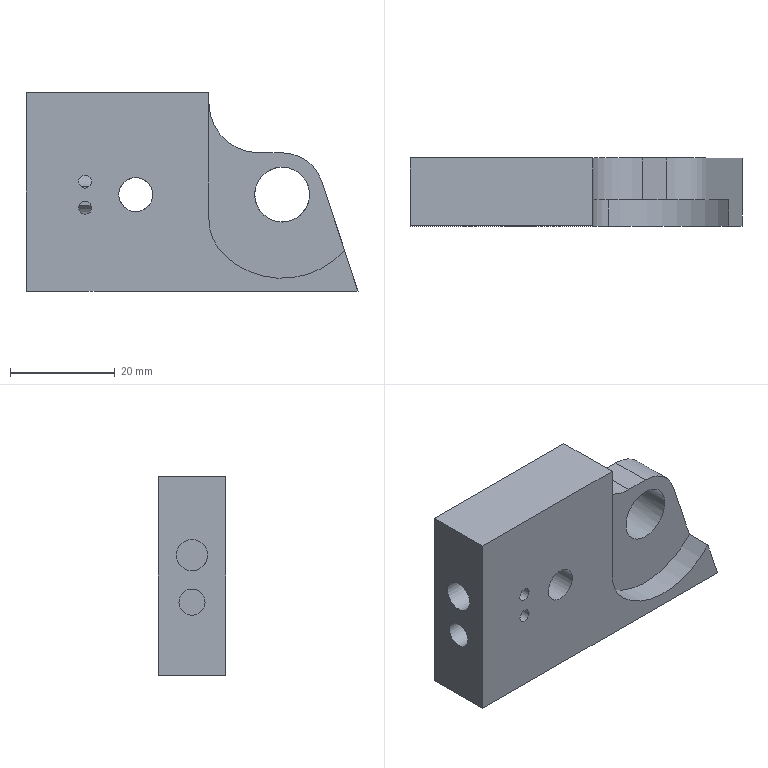Component | NX | BRACKET | 1 solid | 27 faces | volume 21113 mm3 | plane 15 | cylinder 12 | commonest cylinder face diameters 19 x2 2.5 x2 4 x2 16 x1 10.5 x1 32 x1 6.5 x1 6 x1